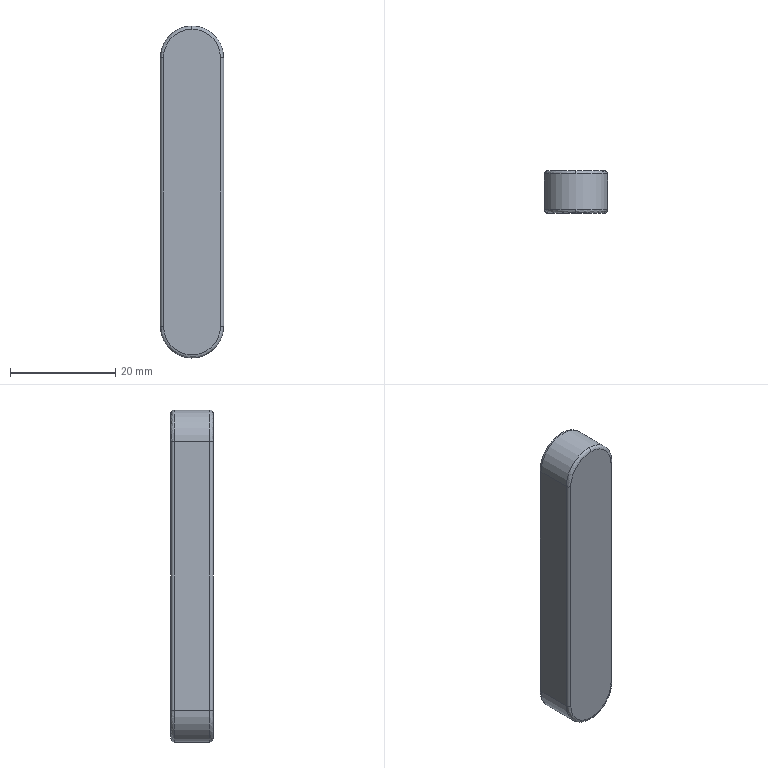Component | SolidWorks | ParallelKey-1 | 1 solid | 17 faces | box 12 x 8 x 63 mm | volume 5779 mm3 | cylinder 7 | spline 6 | plane 4 | commonest cylinder face diameters 1.2 x4 12 x3
STEP:
#1=COLOUR_RGB('',0.7922,0.8196,0.9333);
#2=FILL_AREA_STYLE_COLOUR('',#1);
#3=FILL_AREA_STYLE('',(#2));
#4=SURFACE_STYLE_FILL_AREA(#3);
#5=SURFACE_SIDE_STYLE('',(#4));
#6=SURFACE_STYLE_USAGE(.BOTH.,#5);
#7=PRESENTATION_STYLE_ASSIGNMENT((#6));
#8=CARTESIAN_POINT('',(8.268,9.429,-9.5));
#9=VERTEX_POINT('',#8);
#10=CARTESIAN_POINT('',(8.055,9.429,-9.713));
#11=VERTEX_POINT('',#10);
#12=CARTESIAN_POINT('',(8.268,9.429,-9.5));
#13=CARTESIAN_POINT('',(8.261,9.429,-9.5));
#14=CARTESIAN_POINT('',(8.252,9.429,-9.5));
#15=CARTESIAN_POINT('',(8.24,9.429,-9.502));
#16=CARTESIAN_POINT('',(8.235,9.429,-9.503));
#17=CARTESIAN_POINT('',(8.232,9.429,-9.503));
#18=CARTESIAN_POINT('',(8.231,9.429,-9.503));
#19=CARTESIAN_POINT('',(8.23,9.429,-9.503));
#20=CARTESIAN_POINT('',(8.222,9.429,-9.505));
#21=CARTESIAN_POINT('',(8.212,9.429,-9.507));
#22=CARTESIAN_POINT('',(8.201,9.429,-9.511));
#23=CARTESIAN_POINT('',(8.196,9.429,-9.512));
#24=CARTESIAN_POINT('',(8.193,9.429,-9.514));
#25=CARTESIAN_POINT('',(8.191,9.429,-9.514));
#26=CARTESIAN_POINT('',(8.183,9.429,-9.518));
#27=CARTESIAN_POINT('',(8.173,9.429,-9.522));
#28=CARTESIAN_POINT('',(8.164,9.429,-9.527));
#29=CARTESIAN_POINT('',(8.157,9.429,-9.531));
#30=CARTESIAN_POINT('',(8.154,9.429,-9.533));
#31=CARTESIAN_POINT('',(8.139,9.429,-9.543));
#32=CARTESIAN_POINT('',(8.128,9.429,-9.552));
#33=CARTESIAN_POINT('',(8.112,9.429,-9.567));
#34=CARTESIAN_POINT('',(8.105,9.429,-9.576));
#35=CARTESIAN_POINT('',(8.098,9.429,-9.584));
#36=CARTESIAN_POINT('',(8.094,9.429,-9.59));
#37=CARTESIAN_POINT('',(8.092,9.429,-9.593));
#38=CARTESIAN_POINT('',(8.086,9.429,-9.602));
#39=CARTESIAN_POINT('',(8.08,9.429,-9.612));
#40=CARTESIAN_POINT('',(8.075,9.429,-9.623));
#41=CARTESIAN_POINT('',(8.073,9.429,-9.628));
#42=CARTESIAN_POINT('',(8.071,9.429,-9.631));
#43=CARTESIAN_POINT('',(8.071,9.429,-9.633));
#44=CARTESIAN_POINT('',(8.068,9.429,-9.641));
#45=CARTESIAN_POINT('',(8.064,9.429,-9.65));
#46=CARTESIAN_POINT('',(8.061,9.429,-9.662));
#47=CARTESIAN_POINT('',(8.06,9.429,-9.668));
#48=CARTESIAN_POINT('',(8.059,9.429,-9.671));
#49=CARTESIAN_POINT('',(8.059,9.429,-9.672));
#50=CARTESIAN_POINT('',(8.059,9.429,-9.673));
#51=CARTESIAN_POINT('',(8.056,9.429,-9.687));
#52=CARTESIAN_POINT('',(8.055,9.429,-9.7));
#53=CARTESIAN_POINT('',(8.055,9.429,-9.713));
#54=B_SPLINE_CURVE_WITH_KNOTS('',3,(#12,#13,#14,#15,#16,#17,#18,#19,#20,#21,#22,#23,#24,#25,#26,#27,#28,#29,#30,#31,#32,#33,#34,#35,#36,#37,#38,#39,#40,#41,#42,#43,#44,#45,#46,#47,#48,#49,#50,#51,#52,#53),.UNSPECIFIED.,.F.,.F.,(4,1,1,1,2,2,1,1,2,2,1,2,2,2,1,2,2,1,1,2,2,1,1,1,2,2,4),(0.,0.0625,0.09375,0.1094,0.1172,0.125,0.1875,0.2188,0.2344,0.25,0.3125,0.3438,0.375,0.5,0.5625,0.5938,0.625,0.6875,0.7188,0.7344,0.75,0.8125,0.8438,0.8594,0.8672,0.875,1.),.UNSPECIFIED.);
#55=EDGE_CURVE('',#9,#11,#54,.T.);
#56=ORIENTED_EDGE('',*,*,#55,.F.);
#57=CARTESIAN_POINT('',(8.268,9.453,-9.476));
#58=VERTEX_POINT('',#57);
#59=CARTESIAN_POINT('',(8.268,9.453,-9.5));
#60=DIRECTION('',(-1.,-0.,0.));
#61=DIRECTION('',(0.,0.,1.));
#62=AXIS2_PLACEMENT_3D('',#59,#60,#61);
#63=CIRCLE('',#62,0.02362);
#64=EDGE_CURVE('',#9,#58,#63,.T.);
#65=ORIENTED_EDGE('',*,*,#64,.T.);
#66=CARTESIAN_POINT('',(8.031,9.453,-9.713));
#67=VERTEX_POINT('',#66);
#68=CARTESIAN_POINT('',(8.268,9.453,-9.713));
#69=DIRECTION('',(0.,-1.,-0.));
#70=DIRECTION('',(0.,0.,1.));
#71=AXIS2_PLACEMENT_3D('',#68,#69,#70);
#72=CIRCLE('',#71,0.2362);
#73=EDGE_CURVE('',#58,#67,#72,.T.);
#74=ORIENTED_EDGE('',*,*,#73,.T.);
#75=CARTESIAN_POINT('',(8.055,9.453,-9.713));
#76=DIRECTION('',(-0.,0.,-1.));
#77=DIRECTION('',(-1.,0.,0.));
#78=AXIS2_PLACEMENT_3D('',#75,#76,#77);
#79=CIRCLE('',#78,0.02362);
#80=EDGE_CURVE('',#11,#67,#79,.T.);
#81=ORIENTED_EDGE('',*,*,#80,.F.);
#82=EDGE_LOOP('',(#56,#65,#74,#81));
#83=FACE_OUTER_BOUND('',#82,.T.);
#84=CARTESIAN_POINT('',(8.268,9.429,-9.5));
#85=CARTESIAN_POINT('',(8.143,9.429,-9.5));
#86=CARTESIAN_POINT('',(8.055,9.429,-9.588));
#87=CARTESIAN_POINT('',(8.055,9.429,-9.713));
#88=CARTESIAN_POINT('',(8.268,9.429,-9.486));
#89=CARTESIAN_POINT('',(8.135,9.429,-9.486));
#90=CARTESIAN_POINT('',(8.041,9.429,-9.58));
#91=CARTESIAN_POINT('',(8.041,9.429,-9.713));
#92=CARTESIAN_POINT('',(8.268,9.439,-9.476));
#93=CARTESIAN_POINT('',(8.129,9.439,-9.476));
#94=CARTESIAN_POINT('',(8.031,9.439,-9.574));
#95=CARTESIAN_POINT('',(8.031,9.439,-9.713));
#96=CARTESIAN_POINT('',(8.268,9.453,-9.476));
#97=CARTESIAN_POINT('',(8.129,9.453,-9.476));
#98=CARTESIAN_POINT('',(8.031,9.453,-9.574));
#99=CARTESIAN_POINT('',(8.031,9.453,-9.713));
#100=(BOUNDED_SURFACE()B_SPLINE_SURFACE(3,3,((#84,#85,#86,#87),(#88,#89,#90,#91),(#92,#93,#94,#95),(#96,#97,#98,#99)),.UNSPECIFIED.,.F.,.F.,.F.)B_SPLINE_SURFACE_WITH_KNOTS((4,4),(4,4),(0.,1.),(0.,1.),.UNSPECIFIED.)GEOMETRIC_REPRESENTATION_ITEM()RATIONAL_B_SPLINE_SURFACE(((1.,0.8047,0.8047,1.),(0.8047,0.6476,0.6476,0.8047),(0.8047,0.6476,0.6476,0.8047),(1.,0.8047,0.8047,1.)))REPRESENTATION_ITEM('')SURFACE());
#101=ADVANCED_FACE('',(#83),#100,.T.);
#102=CARTESIAN_POINT('',(8.268,9.72,-9.476));
#103=VERTEX_POINT('',#102);
#104=CARTESIAN_POINT('',(8.031,9.72,-9.713));
#105=VERTEX_POINT('',#104);
#106=CARTESIAN_POINT('',(8.268,9.72,-9.713));
#107=DIRECTION('',(0.,-1.,-0.));
#108=DIRECTION('',(0.,0.,-1.));
#109=AXIS2_PLACEMENT_3D('',#106,#107,#108);
#110=CIRCLE('',#109,0.2362);
#111=EDGE_CURVE('',#103,#105,#110,.T.);
#112=ORIENTED_EDGE('',*,*,#111,.F.);
#113=CARTESIAN_POINT('',(8.268,9.744,-9.5));
#114=VERTEX_POINT('',#113);
#115=CARTESIAN_POINT('',(8.268,9.72,-9.5));
#116=DIRECTION('',(-1.,-0.,0.));
#117=DIRECTION('',(0.,0.,1.));
#118=AXIS2_PLACEMENT_3D('',#115,#116,#117);
#119=CIRCLE('',#118,0.02362);
#120=EDGE_CURVE('',#103,#114,#119,.T.);
#121=ORIENTED_EDGE('',*,*,#120,.T.);
#122=CARTESIAN_POINT('',(8.055,9.744,-9.713));
#123=VERTEX_POINT('',#122);
#124=CARTESIAN_POINT('',(8.268,9.744,-9.5));
#125=CARTESIAN_POINT('',(8.143,9.744,-9.5));
#126=CARTESIAN_POINT('',(8.055,9.744,-9.588));
#127=CARTESIAN_POINT('',(8.055,9.744,-9.713));
#128=(BOUNDED_CURVE()B_SPLINE_CURVE(3,(#124,#125,#126,#127),.UNSPECIFIED.,.F.,.F.)B_SPLINE_CURVE_WITH_KNOTS((4,4),(0.,1.),.UNSPECIFIED.)CURVE()GEOMETRIC_REPRESENTATION_ITEM()RATIONAL_B_SPLINE_CURVE((1.,0.8047,0.8047,1.))REPRESENTATION_ITEM(''));
#129=EDGE_CURVE('',#114,#123,#128,.T.);
#130=ORIENTED_EDGE('',*,*,#129,.T.);
#131=CARTESIAN_POINT('',(8.055,9.72,-9.713));
#132=DIRECTION('',(-0.,0.,-1.));
#133=DIRECTION('',(1.,0.,0.));
#134=AXIS2_PLACEMENT_3D('',#131,#132,#133);
#135=CIRCLE('',#134,0.02362);
#136=EDGE_CURVE('',#105,#123,#135,.T.);
#137=ORIENTED_EDGE('',*,*,#136,.F.);
#138=EDGE_LOOP('',(#112,#121,#130,#137));
#139=FACE_OUTER_BOUND('',#138,.T.);
#140=CARTESIAN_POINT('',(8.268,9.72,-9.476));
#141=CARTESIAN_POINT('',(8.129,9.72,-9.476));
#142=CARTESIAN_POINT('',(8.031,9.72,-9.574));
#143=CARTESIAN_POINT('',(8.031,9.72,-9.713));
#144=CARTESIAN_POINT('',(8.268,9.734,-9.476));
#145=CARTESIAN_POINT('',(8.129,9.734,-9.476));
#146=CARTESIAN_POINT('',(8.031,9.734,-9.574));
#147=CARTESIAN_POINT('',(8.031,9.734,-9.713));
#148=CARTESIAN_POINT('',(8.268,9.744,-9.486));
#149=CARTESIAN_POINT('',(8.135,9.744,-9.486));
#150=CARTESIAN_POINT('',(8.041,9.744,-9.58));
#151=CARTESIAN_POINT('',(8.041,9.744,-9.713));
#152=CARTESIAN_POINT('',(8.268,9.744,-9.5));
#153=CARTESIAN_POINT('',(8.143,9.744,-9.5));
#154=CARTESIAN_POINT('',(8.055,9.744,-9.588));
#155=CARTESIAN_POINT('',(8.055,9.744,-9.713));
#156=(BOUNDED_SURFACE()B_SPLINE_SURFACE(3,3,((#140,#141,#142,#143),(#144,#145,#146,#147),(#148,#149,#150,#151),(#152,#153,#154,#155)),.UNSPECIFIED.,.F.,.F.,.T.)B_SPLINE_SURFACE_WITH_KNOTS((4,4),(4,4),(0.,1.),(0.,1.),.UNSPECIFIED.)GEOMETRIC_REPRESENTATION_ITEM()RATIONAL_B_SPLINE_SURFACE(((1.,0.8047,0.8047,1.),(0.8047,0.6476,0.6476,0.8047),(0.8047,0.6476,0.6476,0.8047),(1.,0.8047,0.8047,1.)))REPRESENTATION_ITEM('')SURFACE());
#157=ADVANCED_FACE('',(#139),#156,.T.);
#158=CARTESIAN_POINT('',(8.268,9.453,-11.957));
#159=VERTEX_POINT('',#158);
#160=CARTESIAN_POINT('',(8.504,9.453,-11.72));
#161=VERTEX_POINT('',#160);
#162=CARTESIAN_POINT('',(8.268,9.453,-11.72));
#163=DIRECTION('',(0.,-1.,-0.));
#164=DIRECTION('',(0.,0.,1.));
#165=AXIS2_PLACEMENT_3D('',#162,#163,#164);
#166=CIRCLE('',#165,0.2362);
#167=EDGE_CURVE('',#159,#161,#166,.T.);
#168=ORIENTED_EDGE('',*,*,#167,.F.);
#169=CARTESIAN_POINT('',(8.268,9.72,-11.957));
#170=VERTEX_POINT('',#169);
#171=CARTESIAN_POINT('',(8.268,9.429,-11.957));
#172=DIRECTION('',(-0.,1.,0.));
#173=VECTOR('',#172,39.37);
#174=LINE('',#171,#173);
#175=EDGE_CURVE('',#159,#170,#174,.T.);
#176=ORIENTED_EDGE('',*,*,#175,.T.);
#177=CARTESIAN_POINT('',(8.504,9.72,-11.72));
#178=VERTEX_POINT('',#177);
#179=CARTESIAN_POINT('',(8.268,9.72,-11.72));
#180=DIRECTION('',(0.,-1.,-0.));
#181=DIRECTION('',(0.,0.,-1.));
#182=AXIS2_PLACEMENT_3D('',#179,#180,#181);
#183=CIRCLE('',#182,0.2362);
#184=EDGE_CURVE('',#170,#178,#183,.T.);
#185=ORIENTED_EDGE('',*,*,#184,.T.);
#186=CARTESIAN_POINT('',(8.504,9.429,-11.72));
#187=DIRECTION('',(0.,-1.,-0.));
#188=VECTOR('',#187,39.37);
#189=LINE('',#186,#188);
#190=EDGE_CURVE('',#178,#161,#189,.T.);
#191=ORIENTED_EDGE('',*,*,#190,.T.);
#192=EDGE_LOOP('',(#168,#176,#185,#191));
#193=FACE_OUTER_BOUND('',#192,.T.);
#194=CARTESIAN_POINT('',(8.268,9.429,-11.72));
#195=DIRECTION('',(-0.,1.,0.));
#196=DIRECTION('',(0.,0.,-1.));
#197=AXIS2_PLACEMENT_3D('',#194,#195,#196);
#198=CYLINDRICAL_SURFACE('',#197,0.2362);
#199=ADVANCED_FACE('',(#193),#198,.T.);
#200=CARTESIAN_POINT('',(8.055,9.429,-11.72));
#201=VERTEX_POINT('',#200);
#202=CARTESIAN_POINT('',(8.055,9.429,-11.72));
#203=DIRECTION('',(-0.,0.,-1.));
#204=VECTOR('',#203,39.37);
#205=LINE('',#202,#204);
#206=EDGE_CURVE('',#11,#201,#205,.T.);
#207=ORIENTED_EDGE('',*,*,#206,.T.);
#208=CARTESIAN_POINT('',(8.48,9.429,-11.72));
#209=VERTEX_POINT('',#208);
#210=CARTESIAN_POINT('',(8.055,9.429,-11.72));
#211=CARTESIAN_POINT('',(8.055,9.429,-11.727));
#212=CARTESIAN_POINT('',(8.056,9.429,-11.737));
#213=CARTESIAN_POINT('',(8.057,9.429,-11.748));
#214=CARTESIAN_POINT('',(8.058,9.429,-11.754));
#215=CARTESIAN_POINT('',(8.058,9.429,-11.756));
#216=CARTESIAN_POINT('',(8.058,9.429,-11.758));
#217=CARTESIAN_POINT('',(8.059,9.429,-11.758));
#218=CARTESIAN_POINT('',(8.06,9.429,-11.766));
#219=CARTESIAN_POINT('',(8.062,9.429,-11.776));
#220=CARTESIAN_POINT('',(8.066,9.429,-11.787));
#221=CARTESIAN_POINT('',(8.068,9.429,-11.792));
#222=CARTESIAN_POINT('',(8.069,9.429,-11.796));
#223=CARTESIAN_POINT('',(8.069,9.429,-11.797));
#224=CARTESIAN_POINT('',(8.073,9.429,-11.805));
#225=CARTESIAN_POINT('',(8.077,9.429,-11.815));
#226=CARTESIAN_POINT('',(8.082,9.429,-11.825));
#227=CARTESIAN_POINT('',(8.086,9.429,-11.831));
#228=CARTESIAN_POINT('',(8.088,9.429,-11.834));
#229=CARTESIAN_POINT('',(8.098,9.429,-11.849));
#230=CARTESIAN_POINT('',(8.107,9.429,-11.86));
#231=CARTESIAN_POINT('',(8.123,9.429,-11.876));
#232=CARTESIAN_POINT('',(8.131,9.429,-11.883));
#233=CARTESIAN_POINT('',(8.139,9.429,-11.89));
#234=CARTESIAN_POINT('',(8.145,9.429,-11.894));
#235=CARTESIAN_POINT('',(8.148,9.429,-11.896));
#236=CARTESIAN_POINT('',(8.157,9.429,-11.902));
#237=CARTESIAN_POINT('',(8.167,9.429,-11.908));
#238=CARTESIAN_POINT('',(8.178,9.429,-11.913));
#239=CARTESIAN_POINT('',(8.183,9.429,-11.915));
#240=CARTESIAN_POINT('',(8.186,9.429,-11.917));
#241=CARTESIAN_POINT('',(8.188,9.429,-11.918));
#242=CARTESIAN_POINT('',(8.196,9.429,-11.921));
#243=CARTESIAN_POINT('',(8.206,9.429,-11.924));
#244=CARTESIAN_POINT('',(8.217,9.429,-11.927));
#245=CARTESIAN_POINT('',(8.223,9.429,-11.928));
#246=CARTESIAN_POINT('',(8.226,9.429,-11.929));
#247=CARTESIAN_POINT('',(8.227,9.429,-11.929));
#248=CARTESIAN_POINT('',(8.228,9.429,-11.929));
#249=CARTESIAN_POINT('',(8.242,9.429,-11.932));
#250=CARTESIAN_POINT('',(8.255,9.429,-11.933));
#251=CARTESIAN_POINT('',(8.274,9.429,-11.933));
#252=CARTESIAN_POINT('',(8.284,9.429,-11.933));
#253=CARTESIAN_POINT('',(8.295,9.429,-11.931));
#254=CARTESIAN_POINT('',(8.301,9.429,-11.93));
#255=CARTESIAN_POINT('',(8.303,9.429,-11.93));
#256=CARTESIAN_POINT('',(8.305,9.429,-11.93));
#257=CARTESIAN_POINT('',(8.306,9.429,-11.93));
#258=CARTESIAN_POINT('',(8.313,9.429,-11.928));
#259=CARTESIAN_POINT('',(8.323,9.429,-11.926));
#260=CARTESIAN_POINT('',(8.335,9.429,-11.922));
#261=CARTESIAN_POINT('',(8.34,9.429,-11.921));
#262=CARTESIAN_POINT('',(8.343,9.429,-11.919));
#263=CARTESIAN_POINT('',(8.344,9.429,-11.919));
#264=CARTESIAN_POINT('',(8.353,9.429,-11.916));
#265=CARTESIAN_POINT('',(8.362,9.429,-11.911));
#266=CARTESIAN_POINT('',(8.372,9.429,-11.906));
#267=CARTESIAN_POINT('',(8.378,9.429,-11.902));
#268=CARTESIAN_POINT('',(8.381,9.429,-11.9));
#269=CARTESIAN_POINT('',(8.396,9.429,-11.89));
#270=CARTESIAN_POINT('',(8.408,9.429,-11.881));
#271=CARTESIAN_POINT('',(8.423,9.429,-11.866));
#272=CARTESIAN_POINT('',(8.431,9.429,-11.857));
#273=CARTESIAN_POINT('',(8.437,9.429,-11.849));
#274=CARTESIAN_POINT('',(8.442,9.429,-11.843));
#275=CARTESIAN_POINT('',(8.444,9.429,-11.84));
#276=CARTESIAN_POINT('',(8.45,9.429,-11.831));
#277=CARTESIAN_POINT('',(8.455,9.429,-11.822));
#278=CARTESIAN_POINT('',(8.46,9.429,-11.81));
#279=CARTESIAN_POINT('',(8.463,9.429,-11.805));
#280=CARTESIAN_POINT('',(8.464,9.429,-11.802));
#281=CARTESIAN_POINT('',(8.465,9.429,-11.8));
#282=CARTESIAN_POINT('',(8.468,9.429,-11.792));
#283=CARTESIAN_POINT('',(8.471,9.429,-11.783));
#284=CARTESIAN_POINT('',(8.474,9.429,-11.771));
#285=CARTESIAN_POINT('',(8.476,9.429,-11.765));
#286=CARTESIAN_POINT('',(8.476,9.429,-11.763));
#287=CARTESIAN_POINT('',(8.476,9.429,-11.761));
#288=CARTESIAN_POINT('',(8.477,9.429,-11.76));
#289=CARTESIAN_POINT('',(8.479,9.429,-11.746));
#290=CARTESIAN_POINT('',(8.48,9.429,-11.733));
#291=CARTESIAN_POINT('',(8.48,9.429,-11.72));
#292=B_SPLINE_CURVE_WITH_KNOTS('',3,(#210,#211,#212,#213,#214,#215,#216,#217,#218,#219,#220,#221,#222,#223,#224,#225,#226,#227,#228,#229,#230,#231,#232,#233,#234,#235,#236,#237,#238,#239,#240,#241,#242,#243,#244,#245,#246,#247,#248,#249,#250,#251,#252,#253,#254,#255,#256,#257,#258,#259,#260,#261,#262,#263,#264,#265,#266,#267,#268,#269,#270,#271,#272,#273,#274,#275,#276,#277,#278,#279,#280,#281,#282,#283,#284,#285,#286,#287,#288,#289,#290,#291),.UNSPECIFIED.,.F.,.F.,(4,1,1,1,2,2,1,1,2,2,1,2,2,2,1,2,2,1,1,2,2,1,1,1,2,2,2,1,1,1,2,2,1,1,2,2,1,2,2,2,1,2,2,1,1,2,2,1,1,1,2,2,4),(0.,0.03125,0.04687,0.05469,0.05859,0.0625,0.09375,0.1094,0.1172,0.125,0.1562,0.1719,0.1875,0.25,0.2812,0.2969,0.3125,0.3437,0.3594,0.3672,0.375,0.4062,0.4219,0.4297,0.4336,0.4375,0.5,0.5312,0.5469,0.5547,0.5586,0.5625,0.5937,0.6094,0.6172,0.625,0.6562,0.6719,0.6875,0.75,0.7813,0.7969,0.8125,0.8438,0.8594,0.8672,0.875,0.9063,0.9219,0.9297,0.9336,0.9375,1.),.UNSPECIFIED.);
#293=EDGE_CURVE('',#201,#209,#292,.T.);
#294=ORIENTED_EDGE('',*,*,#293,.T.);
#295=CARTESIAN_POINT('',(8.48,9.429,-9.713));
#296=VERTEX_POINT('',#295);
#297=CARTESIAN_POINT('',(8.48,9.429,-11.72));
#298=DIRECTION('',(0.,-0.,1.));
#299=VECTOR('',#298,39.37);
#300=LINE('',#297,#299);
#301=EDGE_CURVE('',#209,#296,#300,.T.);
#302=ORIENTED_EDGE('',*,*,#301,.T.);
#303=CARTESIAN_POINT('',(8.48,9.429,-9.713));
#304=CARTESIAN_POINT('',(8.48,9.429,-9.706));
#305=CARTESIAN_POINT('',(8.48,9.429,-9.696));
#306=CARTESIAN_POINT('',(8.479,9.429,-9.685));
#307=CARTESIAN_POINT('',(8.478,9.429,-9.68));
#308=CARTESIAN_POINT('',(8.477,9.429,-9.677));
#309=CARTESIAN_POINT('',(8.477,9.429,-9.676));
#310=CARTESIAN_POINT('',(8.477,9.429,-9.675));
#311=CARTESIAN_POINT('',(8.476,9.429,-9.667));
#312=CARTESIAN_POINT('',(8.473,9.429,-9.657));
#313=CARTESIAN_POINT('',(8.47,9.429,-9.646));
#314=CARTESIAN_POINT('',(8.468,9.429,-9.641));
#315=CARTESIAN_POINT('',(8.467,9.429,-9.638));
#316=CARTESIAN_POINT('',(8.466,9.429,-9.636));
#317=CARTESIAN_POINT('',(8.463,9.429,-9.628));
#318=CARTESIAN_POINT('',(8.458,9.429,-9.618));
#319=CARTESIAN_POINT('',(8.453,9.429,-9.609));
#320=CARTESIAN_POINT('',(8.45,9.429,-9.602));
#321=CARTESIAN_POINT('',(8.448,9.429,-9.599));
#322=CARTESIAN_POINT('',(8.438,9.429,-9.584));
#323=CARTESIAN_POINT('',(8.428,9.429,-9.573));
#324=CARTESIAN_POINT('',(8.413,9.429,-9.557));
#325=CARTESIAN_POINT('',(8.405,9.429,-9.55));
#326=CARTESIAN_POINT('',(8.396,9.429,-9.543));
#327=CARTESIAN_POINT('',(8.39,9.429,-9.539));
#328=CARTESIAN_POINT('',(8.387,9.429,-9.537));
#329=CARTESIAN_POINT('',(8.378,9.429,-9.531));
#330=CARTESIAN_POINT('',(8.369,9.429,-9.525));
#331=CARTESIAN_POINT('',(8.358,9.429,-9.52));
#332=CARTESIAN_POINT('',(8.353,9.429,-9.518));
#333=CARTESIAN_POINT('',(8.349,9.429,-9.516));
#334=CARTESIAN_POINT('',(8.348,9.429,-9.516));
#335=CARTESIAN_POINT('',(8.34,9.429,-9.512));
#336=CARTESIAN_POINT('',(8.33,9.429,-9.509));
#337=CARTESIAN_POINT('',(8.318,9.429,-9.506));
#338=CARTESIAN_POINT('',(8.312,9.429,-9.505));
#339=CARTESIAN_POINT('',(8.31,9.429,-9.504));
#340=CARTESIAN_POINT('',(8.308,9.429,-9.504));
#341=CARTESIAN_POINT('',(8.307,9.429,-9.504));
#342=CARTESIAN_POINT('',(8.294,9.429,-9.501));
#343=CARTESIAN_POINT('',(8.281,9.429,-9.5));
#344=CARTESIAN_POINT('',(8.268,9.429,-9.5));
#345=B_SPLINE_CURVE_WITH_KNOTS('',3,(#303,#304,#305,#306,#307,#308,#309,#310,#311,#312,#313,#314,#315,#316,#317,#318,#319,#320,#321,#322,#323,#324,#325,#326,#327,#328,#329,#330,#331,#332,#333,#334,#335,#336,#337,#338,#339,#340,#341,#342,#343,#344),.UNSPECIFIED.,.F.,.F.,(4,1,1,1,2,2,1,1,2,2,1,2,2,2,1,2,2,1,1,2,2,1,1,1,2,2,4),(0.,0.0625,0.09375,0.1094,0.1172,0.125,0.1875,0.2187,0.2344,0.25,0.3125,0.3437,0.375,0.5,0.5625,0.5937,0.625,0.6875,0.7187,0.7344,0.75,0.8125,0.8437,0.8594,0.8672,0.875,1.),.UNSPECIFIED.);
#346=EDGE_CURVE('',#296,#9,#345,.T.);
#347=ORIENTED_EDGE('',*,*,#346,.T.);
#348=ORIENTED_EDGE('',*,*,#55,.T.);
#349=EDGE_LOOP('',(#207,#294,#302,#347,#348));
#350=FACE_OUTER_BOUND('',#349,.T.);
#351=CARTESIAN_POINT('',(8.268,9.429,-11.72));
#352=DIRECTION('',(0.,-1.,-0.));
#353=DIRECTION('',(0.,-0.,1.));
#354=AXIS2_PLACEMENT_3D('',#351,#352,#353);
#355=PLANE('',#354);
#356=ADVANCED_FACE('',(#350),#355,.T.);
#357=CARTESIAN_POINT('',(8.48,9.453,-11.72));
#358=DIRECTION('',(-0.,0.,-1.));
#359=DIRECTION('',(1.,0.,0.));
#360=AXIS2_PLACEMENT_3D('',#357,#358,#359);
#361=CIRCLE('',#360,0.02362);
#362=EDGE_CURVE('',#161,#209,#361,.T.);
#363=ORIENTED_EDGE('',*,*,#362,.T.);
#364=ORIENTED_EDGE('',*,*,#293,.F.);
#365=CARTESIAN_POINT('',(8.031,9.453,-11.72));
#366=VERTEX_POINT('',#365);
#367=CARTESIAN_POINT('',(8.055,9.453,-11.72));
#368=DIRECTION('',(-0.,0.,-1.));
#369=DIRECTION('',(-1.,0.,0.));
#370=AXIS2_PLACEMENT_3D('',#367,#368,#369);
#371=CIRCLE('',#370,0.02362);
#372=EDGE_CURVE('',#201,#366,#371,.T.);
#373=ORIENTED_EDGE('',*,*,#372,.T.);
#374=CARTESIAN_POINT('',(8.268,9.453,-11.72));
#375=DIRECTION('',(0.,-1.,-0.));
#376=DIRECTION('',(0.,0.,1.));
#377=AXIS2_PLACEMENT_3D('',#374,#375,#376);
#378=CIRCLE('',#377,0.2362);
#379=EDGE_CURVE('',#366,#159,#378,.T.);
#380=ORIENTED_EDGE('',*,*,#379,.T.);
#381=ORIENTED_EDGE('',*,*,#167,.T.);
#382=EDGE_LOOP('',(#363,#364,#373,#380,#381));
#383=FACE_OUTER_BOUND('',#382,.T.);
#384=CARTESIAN_POINT('',(8.055,9.429,-11.72));
#385=CARTESIAN_POINT('',(8.055,9.429,-12.146));
#386=CARTESIAN_POINT('',(8.48,9.429,-12.146));
#387=CARTESIAN_POINT('',(8.48,9.429,-11.72));
#388=CARTESIAN_POINT('',(8.041,9.429,-11.72));
#389=CARTESIAN_POINT('',(8.041,9.429,-12.173));
#390=CARTESIAN_POINT('',(8.494,9.429,-12.173));
#391=CARTESIAN_POINT('',(8.494,9.429,-11.72));
#392=CARTESIAN_POINT('',(8.031,9.439,-11.72));
#393=CARTESIAN_POINT('',(8.031,9.439,-12.193));
#394=CARTESIAN_POINT('',(8.504,9.439,-12.193));
#395=CARTESIAN_POINT('',(8.504,9.439,-11.72));
#396=CARTESIAN_POINT('',(8.031,9.453,-11.72));
#397=CARTESIAN_POINT('',(8.031,9.453,-12.193));
#398=CARTESIAN_POINT('',(8.504,9.453,-12.193));
#399=CARTESIAN_POINT('',(8.504,9.453,-11.72));
#400=(BOUNDED_SURFACE()B_SPLINE_SURFACE(3,3,((#384,#385,#386,#387),(#388,#389,#390,#391),(#392,#393,#394,#395),(#396,#397,#398,#399)),.UNSPECIFIED.,.F.,.F.,.T.)B_SPLINE_SURFACE_WITH_KNOTS((4,4),(4,4),(0.,1.),(0.,1.),.UNSPECIFIED.)GEOMETRIC_REPRESENTATION_ITEM()RATIONAL_B_SPLINE_SURFACE(((1.,0.3333,0.3333,1.),(0.8047,0.2682,0.2682,0.8047),(0.8047,0.2682,0.2682,0.8047),(1.,0.3333,0.3333,1.)))REPRESENTATION_ITEM('')SURFACE());
#401=ADVANCED_FACE('',(#383),#400,.T.);
#402=ORIENTED_EDGE('',*,*,#80,.T.);
#403=CARTESIAN_POINT('',(8.031,9.453,-11.72));
#404=DIRECTION('',(-0.,0.,-1.));
#405=VECTOR('',#404,39.37);
#406=LINE('',#403,#405);
#407=EDGE_CURVE('',#67,#366,#406,.T.);
#408=ORIENTED_EDGE('',*,*,#407,.T.);
#409=ORIENTED_EDGE('',*,*,#372,.F.);
#410=ORIENTED_EDGE('',*,*,#206,.F.);
#411=EDGE_LOOP('',(#402,#408,#409,#410));
#412=FACE_OUTER_BOUND('',#411,.T.);
#413=CARTESIAN_POINT('',(8.055,9.453,-11.72));
#414=DIRECTION('',(0.,-0.,1.));
#415=DIRECTION('',(-1.,0.,0.));
#416=AXIS2_PLACEMENT_3D('',#413,#414,#415);
#417=CYLINDRICAL_SURFACE('',#416,0.02362);
#418=ADVANCED_FACE('',(#412),#417,.T.);
#419=ORIENTED_EDGE('',*,*,#64,.F.);
#420=ORIENTED_EDGE('',*,*,#346,.F.);
#421=CARTESIAN_POINT('',(8.504,9.453,-9.713));
#422=VERTEX_POINT('',#421);
#423=CARTESIAN_POINT('',(8.48,9.453,-9.713));
#424=DIRECTION('',(0.,-0.,1.));
#425=DIRECTION('',(1.,0.,0.));
#426=AXIS2_PLACEMENT_3D('',#423,#424,#425);
#427=CIRCLE('',#426,0.02362);
#428=EDGE_CURVE('',#296,#422,#427,.T.);
#429=ORIENTED_EDGE('',*,*,#428,.T.);
#430=CARTESIAN_POINT('',(8.268,9.453,-9.713));
#431=DIRECTION('',(0.,-1.,-0.));
#432=DIRECTION('',(0.,0.,1.));
#433=AXIS2_PLACEMENT_3D('',#430,#431,#432);
#434=CIRCLE('',#433,0.2362);
#435=EDGE_CURVE('',#422,#58,#434,.T.);
#436=ORIENTED_EDGE('',*,*,#435,.T.);
#437=EDGE_LOOP('',(#419,#420,#429,#436));
#438=FACE_OUTER_BOUND('',#437,.T.);
#439=CARTESIAN_POINT('',(8.48,9.429,-9.713));
#440=CARTESIAN_POINT('',(8.48,9.429,-9.588));
#441=CARTESIAN_POINT('',(8.392,9.429,-9.5));
#442=CARTESIAN_POINT('',(8.268,9.429,-9.5));
#443=CARTESIAN_POINT('',(8.494,9.429,-9.713));
#444=CARTESIAN_POINT('',(8.494,9.429,-9.58));
#445=CARTESIAN_POINT('',(8.4,9.429,-9.486));
#446=CARTESIAN_POINT('',(8.268,9.429,-9.486));
#447=CARTESIAN_POINT('',(8.504,9.439,-9.713));
#448=CARTESIAN_POINT('',(8.504,9.439,-9.574));
#449=CARTESIAN_POINT('',(8.406,9.439,-9.476));
#450=CARTESIAN_POINT('',(8.268,9.439,-9.476));
#451=CARTESIAN_POINT('',(8.504,9.453,-9.713));
#452=CARTESIAN_POINT('',(8.504,9.453,-9.574));
#453=CARTESIAN_POINT('',(8.406,9.453,-9.476));
#454=CARTESIAN_POINT('',(8.268,9.453,-9.476));
#455=(BOUNDED_SURFACE()B_SPLINE_SURFACE(3,3,((#439,#440,#441,#442),(#443,#444,#445,#446),(#447,#448,#449,#450),(#451,#452,#453,#454)),.UNSPECIFIED.,.F.,.F.,.T.)B_SPLINE_SURFACE_WITH_KNOTS((4,4),(4,4),(0.,1.),(0.,1.),.UNSPECIFIED.)GEOMETRIC_REPRESENTATION_ITEM()RATIONAL_B_SPLINE_SURFACE(((1.,0.8047,0.8047,1.),(0.8047,0.6476,0.6476,0.8047),(0.8047,0.6476,0.6476,0.8047),(1.,0.8047,0.8047,1.)))REPRESENTATION_ITEM('')SURFACE());
#456=ADVANCED_FACE('',(#438),#455,.T.);
#457=ORIENTED_EDGE('',*,*,#428,.F.);
#458=ORIENTED_EDGE('',*,*,#301,.F.);
#459=ORIENTED_EDGE('',*,*,#362,.F.);
#460=CARTESIAN_POINT('',(8.504,9.453,-11.72));
#461=DIRECTION('',(0.,-0.,1.));
#462=VECTOR('',#461,39.37);
#463=LINE('',#460,#462);
#464=EDGE_CURVE('',#161,#422,#463,.T.);
#465=ORIENTED_EDGE('',*,*,#464,.T.);
#466=EDGE_LOOP('',(#457,#458,#459,#465));
#467=FACE_OUTER_BOUND('',#466,.T.);
#468=CARTESIAN_POINT('',(8.48,9.453,-11.72));
#469=DIRECTION('',(-0.,0.,-1.));
#470=DIRECTION('',(1.,0.,0.));
#471=AXIS2_PLACEMENT_3D('',#468,#469,#470);
#472=CYLINDRICAL_SURFACE('',#471,0.02362);
#473=ADVANCED_FACE('',(#467),#472,.T.);
#474=ORIENTED_EDGE('',*,*,#175,.F.);
#475=ORIENTED_EDGE('',*,*,#379,.F.);
#476=CARTESIAN_POINT('',(8.031,9.72,-11.72));
#477=VERTEX_POINT('',#476);
#478=CARTESIAN_POINT('',(8.031,9.429,-11.72));
#479=DIRECTION('',(-0.,1.,0.));
#480=VECTOR('',#479,39.37);
#481=LINE('',#478,#480);
#482=EDGE_CURVE('',#366,#477,#481,.T.);
#483=ORIENTED_EDGE('',*,*,#482,.T.);
#484=CARTESIAN_POINT('',(8.268,9.72,-11.72));
#485=DIRECTION('',(0.,-1.,-0.));
#486=DIRECTION('',(0.,0.,-1.));
#487=AXIS2_PLACEMENT_3D('',#484,#485,#486);
#488=CIRCLE('',#487,0.2362);
#489=EDGE_CURVE('',#477,#170,#488,.T.);
#490=ORIENTED_EDGE('',*,*,#489,.T.);
#491=EDGE_LOOP('',(#474,#475,#483,#490));
#492=FACE_OUTER_BOUND('',#491,.T.);
#493=CARTESIAN_POINT('',(8.268,9.429,-11.72));
#494=DIRECTION('',(-0.,1.,0.));
#495=DIRECTION('',(0.,0.,-1.));
#496=AXIS2_PLACEMENT_3D('',#493,#494,#495);
#497=CYLINDRICAL_SURFACE('',#496,0.2362);
#498=ADVANCED_FACE('',(#492),#497,.T.);
#499=ORIENTED_EDGE('',*,*,#407,.F.);
#500=CARTESIAN_POINT('',(8.031,9.429,-9.713));
#501=DIRECTION('',(0.,-1.,-0.));
#502=VECTOR('',#501,39.37);
#503=LINE('',#500,#502);
#504=EDGE_CURVE('',#105,#67,#503,.T.);
#505=ORIENTED_EDGE('',*,*,#504,.F.);
#506=CARTESIAN_POINT('',(8.031,9.72,-11.72));
#507=DIRECTION('',(0.,-0.,1.));
#508=VECTOR('',#507,39.37);
#509=LINE('',#506,#508);
#510=EDGE_CURVE('',#477,#105,#509,.T.);
#511=ORIENTED_EDGE('',*,*,#510,.F.);
#512=ORIENTED_EDGE('',*,*,#482,.F.);
#513=EDGE_LOOP('',(#499,#505,#511,#512));
#514=FACE_OUTER_BOUND('',#513,.T.);
#515=CARTESIAN_POINT('',(8.031,9.429,-11.72));
#516=DIRECTION('',(1.,0.,-0.));
#517=DIRECTION('',(0.,-0.,1.));
#518=AXIS2_PLACEMENT_3D('',#515,#516,#517);
#519=PLANE('',#518);
#520=ADVANCED_FACE('',(#514),#519,.F.);
#521=CARTESIAN_POINT('',(8.504,9.72,-9.713));
#522=VERTEX_POINT('',#521);
#523=CARTESIAN_POINT('',(8.504,9.429,-9.713));
#524=DIRECTION('',(-0.,1.,0.));
#525=VECTOR('',#524,39.37);
#526=LINE('',#523,#525);
#527=EDGE_CURVE('',#422,#522,#526,.T.);
#528=ORIENTED_EDGE('',*,*,#527,.T.);
#529=CARTESIAN_POINT('',(8.268,9.72,-9.713));
#530=DIRECTION('',(0.,-1.,-0.));
#531=DIRECTION('',(0.,0.,-1.));
#532=AXIS2_PLACEMENT_3D('',#529,#530,#531);
#533=CIRCLE('',#532,0.2362);
#534=EDGE_CURVE('',#522,#103,#533,.T.);
#535=ORIENTED_EDGE('',*,*,#534,.T.);
#536=ORIENTED_EDGE('',*,*,#111,.T.);
#537=ORIENTED_EDGE('',*,*,#504,.T.);
#538=ORIENTED_EDGE('',*,*,#73,.F.);
#539=ORIENTED_EDGE('',*,*,#435,.F.);
#540=EDGE_LOOP('',(#528,#535,#536,#537,#538,#539));
#541=FACE_OUTER_BOUND('',#540,.T.);
#542=CARTESIAN_POINT('',(8.268,9.429,-9.713));
#543=DIRECTION('',(-0.,1.,0.));
#544=DIRECTION('',(0.,0.,-1.));
#545=AXIS2_PLACEMENT_3D('',#542,#543,#544);
#546=CYLINDRICAL_SURFACE('',#545,0.2362);
#547=ADVANCED_FACE('',(#541),#546,.T.);
#548=ORIENTED_EDGE('',*,*,#464,.F.);
#549=ORIENTED_EDGE('',*,*,#190,.F.);
#550=CARTESIAN_POINT('',(8.504,9.72,-11.72));
#551=DIRECTION('',(-0.,0.,-1.));
#552=VECTOR('',#551,39.37);
#553=LINE('',#550,#552);
#554=EDGE_CURVE('',#522,#178,#553,.T.);
#555=ORIENTED_EDGE('',*,*,#554,.F.);
#556=ORIENTED_EDGE('',*,*,#527,.F.);
#557=EDGE_LOOP('',(#548,#549,#555,#556));
#558=FACE_OUTER_BOUND('',#557,.T.);
#559=CARTESIAN_POINT('',(8.504,9.429,-11.72));
#560=DIRECTION('',(-1.,-0.,0.));
#561=DIRECTION('',(-0.,0.,-1.));
#562=AXIS2_PLACEMENT_3D('',#559,#560,#561);
#563=PLANE('',#562);
#564=ADVANCED_FACE('',(#558),#563,.F.);
#565=ORIENTED_EDGE('',*,*,#489,.F.);
#566=CARTESIAN_POINT('',(8.055,9.744,-11.72));
#567=VERTEX_POINT('',#566);
#568=CARTESIAN_POINT('',(8.055,9.72,-11.72));
#569=DIRECTION('',(-0.,0.,-1.));
#570=DIRECTION('',(-1.,0.,0.));
#571=AXIS2_PLACEMENT_3D('',#568,#569,#570);
#572=CIRCLE('',#571,0.02362);
#573=EDGE_CURVE('',#477,#567,#572,.T.);
#574=ORIENTED_EDGE('',*,*,#573,.T.);
#575=CARTESIAN_POINT('',(8.48,9.744,-11.72));
#576=VERTEX_POINT('',#575);
#577=CARTESIAN_POINT('',(8.055,9.744,-11.72));
#578=CARTESIAN_POINT('',(8.055,9.744,-12.146));
#579=CARTESIAN_POINT('',(8.48,9.744,-12.146));
#580=CARTESIAN_POINT('',(8.48,9.744,-11.72));
#581=(BOUNDED_CURVE()B_SPLINE_CURVE(3,(#577,#578,#579,#580),.UNSPECIFIED.,.F.,.F.)B_SPLINE_CURVE_WITH_KNOTS((4,4),(0.,1.),.UNSPECIFIED.)CURVE()GEOMETRIC_REPRESENTATION_ITEM()RATIONAL_B_SPLINE_CURVE((1.,0.3333,0.3333,1.))REPRESENTATION_ITEM(''));
#582=EDGE_CURVE('',#567,#576,#581,.T.);
#583=ORIENTED_EDGE('',*,*,#582,.T.);
#584=CARTESIAN_POINT('',(8.48,9.72,-11.72));
#585=DIRECTION('',(-0.,0.,-1.));
#586=DIRECTION('',(1.,0.,0.));
#587=AXIS2_PLACEMENT_3D('',#584,#585,#586);
#588=CIRCLE('',#587,0.02362);
#589=EDGE_CURVE('',#576,#178,#588,.T.);
#590=ORIENTED_EDGE('',*,*,#589,.T.);
#591=ORIENTED_EDGE('',*,*,#184,.F.);
#592=EDGE_LOOP('',(#565,#574,#583,#590,#591));
#593=FACE_OUTER_BOUND('',#592,.T.);
#594=CARTESIAN_POINT('',(8.031,9.72,-11.72));
#595=CARTESIAN_POINT('',(8.031,9.72,-12.193));
#596=CARTESIAN_POINT('',(8.504,9.72,-12.193));
#597=CARTESIAN_POINT('',(8.504,9.72,-11.72));
#598=CARTESIAN_POINT('',(8.031,9.734,-11.72));
#599=CARTESIAN_POINT('',(8.031,9.734,-12.193));
#600=CARTESIAN_POINT('',(8.504,9.734,-12.193));
#601=CARTESIAN_POINT('',(8.504,9.734,-11.72));
#602=CARTESIAN_POINT('',(8.041,9.744,-11.72));
#603=CARTESIAN_POINT('',(8.041,9.744,-12.173));
#604=CARTESIAN_POINT('',(8.494,9.744,-12.173));
#605=CARTESIAN_POINT('',(8.494,9.744,-11.72));
#606=CARTESIAN_POINT('',(8.055,9.744,-11.72));
#607=CARTESIAN_POINT('',(8.055,9.744,-12.146));
#608=CARTESIAN_POINT('',(8.48,9.744,-12.146));
#609=CARTESIAN_POINT('',(8.48,9.744,-11.72));
#610=(BOUNDED_SURFACE()B_SPLINE_SURFACE(3,3,((#594,#595,#596,#597),(#598,#599,#600,#601),(#602,#603,#604,#605),(#606,#607,#608,#609)),.UNSPECIFIED.,.F.,.F.,.T.)B_SPLINE_SURFACE_WITH_KNOTS((4,4),(4,4),(0.,1.),(0.,1.),.UNSPECIFIED.)GEOMETRIC_REPRESENTATION_ITEM()RATIONAL_B_SPLINE_SURFACE(((1.,0.3333,0.3333,1.),(0.8047,0.2682,0.2682,0.8047),(0.8047,0.2682,0.2682,0.8047),(1.,0.3333,0.3333,1.)))REPRESENTATION_ITEM('')SURFACE());
#611=ADVANCED_FACE('',(#593),#610,.T.);
#612=ORIENTED_EDGE('',*,*,#136,.T.);
#613=CARTESIAN_POINT('',(8.055,9.744,-11.72));
#614=DIRECTION('',(-0.,0.,-1.));
#615=VECTOR('',#614,39.37);
#616=LINE('',#613,#615);
#617=EDGE_CURVE('',#123,#567,#616,.T.);
#618=ORIENTED_EDGE('',*,*,#617,.T.);
#619=ORIENTED_EDGE('',*,*,#573,.F.);
#620=ORIENTED_EDGE('',*,*,#510,.T.);
#621=EDGE_LOOP('',(#612,#618,#619,#620));
#622=FACE_OUTER_BOUND('',#621,.T.);
#623=CARTESIAN_POINT('',(8.055,9.72,-11.72));
#624=DIRECTION('',(-0.,0.,-1.));
#625=DIRECTION('',(1.,0.,0.));
#626=AXIS2_PLACEMENT_3D('',#623,#624,#625);
#627=CYLINDRICAL_SURFACE('',#626,0.02362);
#628=ADVANCED_FACE('',(#622),#627,.T.);
#629=ORIENTED_EDGE('',*,*,#120,.F.);
#630=ORIENTED_EDGE('',*,*,#534,.F.);
#631=CARTESIAN_POINT('',(8.48,9.744,-9.713));
#632=VERTEX_POINT('',#631);
#633=CARTESIAN_POINT('',(8.48,9.72,-9.713));
#634=DIRECTION('',(0.,-0.,1.));
#635=DIRECTION('',(1.,0.,0.));
#636=AXIS2_PLACEMENT_3D('',#633,#634,#635);
#637=CIRCLE('',#636,0.02362);
#638=EDGE_CURVE('',#522,#632,#637,.T.);
#639=ORIENTED_EDGE('',*,*,#638,.T.);
#640=CARTESIAN_POINT('',(8.48,9.744,-9.713));
#641=CARTESIAN_POINT('',(8.48,9.744,-9.588));
#642=CARTESIAN_POINT('',(8.392,9.744,-9.5));
#643=CARTESIAN_POINT('',(8.268,9.744,-9.5));
#644=(BOUNDED_CURVE()B_SPLINE_CURVE(3,(#640,#641,#642,#643),.UNSPECIFIED.,.F.,.T.)B_SPLINE_CURVE_WITH_KNOTS((4,4),(0.,1.),.UNSPECIFIED.)CURVE()GEOMETRIC_REPRESENTATION_ITEM()RATIONAL_B_SPLINE_CURVE((1.,0.8047,0.8047,1.))REPRESENTATION_ITEM(''));
#645=EDGE_CURVE('',#632,#114,#644,.T.);
#646=ORIENTED_EDGE('',*,*,#645,.T.);
#647=EDGE_LOOP('',(#629,#630,#639,#646));
#648=FACE_OUTER_BOUND('',#647,.T.);
#649=CARTESIAN_POINT('',(8.504,9.72,-9.713));
#650=CARTESIAN_POINT('',(8.504,9.72,-9.574));
#651=CARTESIAN_POINT('',(8.406,9.72,-9.476));
#652=CARTESIAN_POINT('',(8.268,9.72,-9.476));
#653=CARTESIAN_POINT('',(8.504,9.734,-9.713));
#654=CARTESIAN_POINT('',(8.504,9.734,-9.574));
#655=CARTESIAN_POINT('',(8.406,9.734,-9.476));
#656=CARTESIAN_POINT('',(8.268,9.734,-9.476));
#657=CARTESIAN_POINT('',(8.494,9.744,-9.713));
#658=CARTESIAN_POINT('',(8.494,9.744,-9.58));
#659=CARTESIAN_POINT('',(8.4,9.744,-9.486));
#660=CARTESIAN_POINT('',(8.268,9.744,-9.486));
#661=CARTESIAN_POINT('',(8.48,9.744,-9.713));
#662=CARTESIAN_POINT('',(8.48,9.744,-9.588));
#663=CARTESIAN_POINT('',(8.392,9.744,-9.5));
#664=CARTESIAN_POINT('',(8.268,9.744,-9.5));
#665=(BOUNDED_SURFACE()B_SPLINE_SURFACE(3,3,((#649,#650,#651,#652),(#653,#654,#655,#656),(#657,#658,#659,#660),(#661,#662,#663,#664)),.UNSPECIFIED.,.F.,.F.,.F.)B_SPLINE_SURFACE_WITH_KNOTS((4,4),(4,4),(0.,1.),(0.,1.),.UNSPECIFIED.)GEOMETRIC_REPRESENTATION_ITEM()RATIONAL_B_SPLINE_SURFACE(((1.,0.8047,0.8047,1.),(0.8047,0.6476,0.6476,0.8047),(0.8047,0.6476,0.6476,0.8047),(1.,0.8047,0.8047,1.)))REPRESENTATION_ITEM('')SURFACE());
#666=ADVANCED_FACE('',(#648),#665,.T.);
#667=ORIENTED_EDGE('',*,*,#638,.F.);
#668=ORIENTED_EDGE('',*,*,#554,.T.);
#669=ORIENTED_EDGE('',*,*,#589,.F.);
#670=CARTESIAN_POINT('',(8.48,9.744,-11.72));
#671=DIRECTION('',(0.,-0.,1.));
#672=VECTOR('',#671,39.37);
#673=LINE('',#670,#672);
#674=EDGE_CURVE('',#576,#632,#673,.T.);
#675=ORIENTED_EDGE('',*,*,#674,.T.);
#676=EDGE_LOOP('',(#667,#668,#669,#675));
#677=FACE_OUTER_BOUND('',#676,.T.);
#678=CARTESIAN_POINT('',(8.48,9.72,-11.72));
#679=DIRECTION('',(0.,-0.,1.));
#680=DIRECTION('',(-1.,0.,0.));
#681=AXIS2_PLACEMENT_3D('',#678,#679,#680);
#682=CYLINDRICAL_SURFACE('',#681,0.02362);
#683=ADVANCED_FACE('',(#677),#682,.T.);
#684=ORIENTED_EDGE('',*,*,#129,.F.);
#685=ORIENTED_EDGE('',*,*,#645,.F.);
#686=ORIENTED_EDGE('',*,*,#674,.F.);
#687=ORIENTED_EDGE('',*,*,#582,.F.);
#688=ORIENTED_EDGE('',*,*,#617,.F.);
#689=EDGE_LOOP('',(#684,#685,#686,#687,#688));
#690=FACE_OUTER_BOUND('',#689,.T.);
#691=CARTESIAN_POINT('',(8.268,9.744,-11.72));
#692=DIRECTION('',(0.,-1.,-0.));
#693=DIRECTION('',(0.,-0.,1.));
#694=AXIS2_PLACEMENT_3D('',#691,#692,#693);
#695=PLANE('',#694);
#696=ADVANCED_FACE('',(#690),#695,.F.);
#697=CLOSED_SHELL('',(#101,#157,#199,#356,#401,#418,#456,#473,#498,#520,#547,#564,#611,#628,#666,#683,#696));
#698=MANIFOLD_SOLID_BREP('',#697);
#699=STYLED_ITEM('',(#7),#698);
#700=PRESENTATION_LAYER_ASSIGNMENT('','',(#699));
#701=CARTESIAN_POINT('',(0.,0.,0.));
#702=DIRECTION('',(0.,0.,1.));
#703=DIRECTION('',(1.,0.,0.));
#704=AXIS2_PLACEMENT_3D('',#701,#702,#703);
#705=(LENGTH_UNIT()NAMED_UNIT(*)SI_UNIT($,.METRE.));
#706=LENGTH_MEASURE_WITH_UNIT(LENGTH_MEASURE(0.0254),#705);
#707=DIMENSIONAL_EXPONENTS(1.,0.,0.,0.,0.,0.,0.);
#708=(CONVERSION_BASED_UNIT('',#706)LENGTH_UNIT()NAMED_UNIT(#707));
#709=UNCERTAINTY_MEASURE_WITH_UNIT(LENGTH_MEASURE(0.00001),#708,'','');
#710=(NAMED_UNIT(*)PLANE_ANGLE_UNIT()SI_UNIT($,.RADIAN.));
#711=(NAMED_UNIT(*)SI_UNIT($,.STERADIAN.)SOLID_ANGLE_UNIT());
#712=(GEOMETRIC_REPRESENTATION_CONTEXT(3)GLOBAL_UNCERTAINTY_ASSIGNED_CONTEXT((#709))GLOBAL_UNIT_ASSIGNED_CONTEXT((#708,#710,#711))REPRESENTATION_CONTEXT('',''));
#713=ADVANCED_BREP_SHAPE_REPRESENTATION('',(#698,#704),#712);
#714=(LENGTH_UNIT()NAMED_UNIT(*)SI_UNIT($,.METRE.));
#715=LENGTH_MEASURE_WITH_UNIT(LENGTH_MEASURE(0.0254),#714);
#716=DIMENSIONAL_EXPONENTS(1.,0.,0.,0.,0.,0.,0.);
#717=(CONVERSION_BASED_UNIT('',#715)LENGTH_UNIT()NAMED_UNIT(#716));
#718=UNCERTAINTY_MEASURE_WITH_UNIT(LENGTH_MEASURE(0.00001),#717,'','');
#719=(NAMED_UNIT(*)PLANE_ANGLE_UNIT()SI_UNIT($,.RADIAN.));
#720=(NAMED_UNIT(*)SI_UNIT($,.STERADIAN.)SOLID_ANGLE_UNIT());
#721=(GEOMETRIC_REPRESENTATION_CONTEXT(3)GLOBAL_UNCERTAINTY_ASSIGNED_CONTEXT((#718))GLOBAL_UNIT_ASSIGNED_CONTEXT((#717,#719,#720))REPRESENTATION_CONTEXT('',''));
#722=MECHANICAL_DESIGN_GEOMETRIC_PRESENTATION_REPRESENTATION('',(#699),#721);